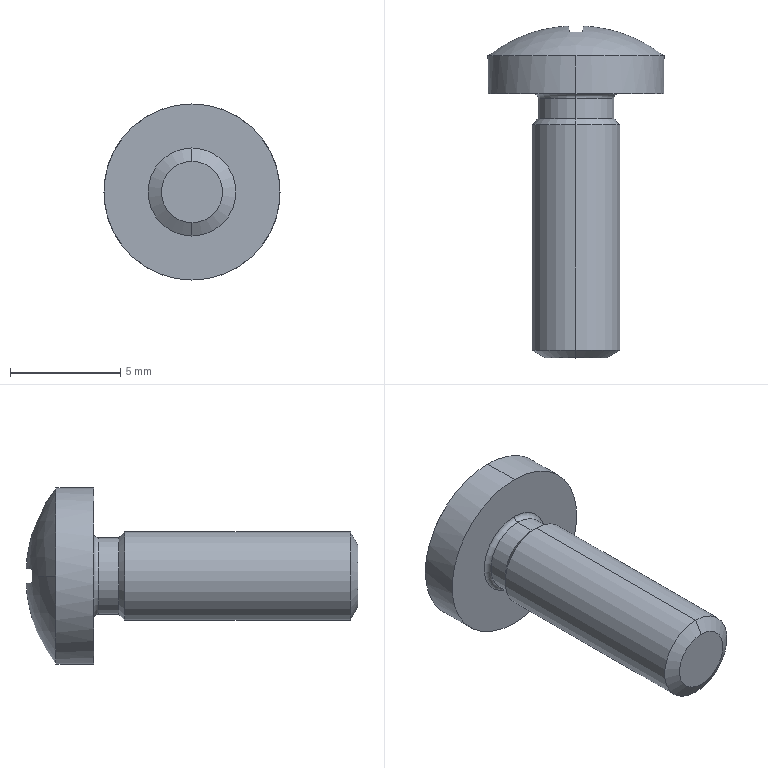Component | SolidWorks | GB_T818-2000PhillipsPanHeadScrewM4_12-1 | 1 solid | 28 faces | box 8 x 15.08 x 8 mm | volume 264 mm3 | plane 14 | cylinder 6 | cone 4 | torus 2 | sphere 2 | commonest cylinder face diameters 3.464 x2 8 x2 4 x2
build123d program:
from build123d import *


with BuildPart() as part:
    # Sketch2 → Base-Revolve (revolve)
    with BuildSketch(Plane.XY, mode=Mode.PRIVATE) as base_revolve_sk:
        with BuildLine():
            Line((0, 0), (15.1, 0))
            Line((15.1, 0), (15.1, 2))
            Line((15.1, 2), (4.5, 2))
            Line((4.5, 2), (4.232, 1.732))
            Line((4.232, 1.732), (3.318, 1.732))
            ThreePointArc((3.318, 1.732), (3.164, 1.796), (3.1, 1.95))
            Line((3.1, 1.95), (3.1, 4))
            Line((3.1, 4), (1.377, 4))
            ThreePointArc((1.377, 4), (0.3538, 2.115), (0, 0))
        make_face()
    revolve(base_revolve_sk.sketch.rotate(Axis((-1.332, 0, 0), (1, 0, 0)), 90), axis=Axis((-1.332, 0, 0), (1, 0, 0)))

    # Sketch3 → Cut-Revolve1 (revolve, cut)
    with BuildSketch(Plane.XY, mode=Mode.PRIVATE) as cut_revolve1_sk:
        Polygon((14.754, 2), (15.454, 2), (15.1, 1.394), align=None)
    revolve(cut_revolve1_sk.sketch.rotate(Axis((-0.2428, 0, 0), (1, 0, 0)), 90), axis=Axis((-0.2428, 0, 0), (1, 0, 0)), mode=Mode.SUBTRACT)

    # Sketch5 → Cut-Loft1 section 0
    with BuildSketch(Plane(origin=(0, 0, 0), x_dir=(0, 0, -1), z_dir=(1, 0, 0)), mode=Mode.PRIVATE) as cut_loft1_s0:
        with BuildLine():
            Line((0.35, 2.2), (-0.35, 2.2))
            Line((-0.35, 2.2), (-0.35, -2.2))
            Line((-0.35, -2.2), (0.35, -2.2))
            Line((0.35, -2.2), (0.35, 2.2))
        make_face()
    cut_loft1 = loft([Vertex(2.4, 0, 0), cut_loft1_s0.sketch], mode=Mode.SUBTRACT)

    # Mirror1: Cut-Loft1 across plane
    add(cut_loft1.mirror(Plane(origin=(0, 0, 0), x_dir=(0, 0.7071, 0.7071), z_dir=(0, -0.7071, 0.7071))), mode=Mode.SUBTRACT)


solid = part.part

# Placed as in the assembly
solid = solid.moved(Location((-112.444, 119.266, -150.597), (0, 0, -90)))
STEP:
#1=COLOUR_RGB('',0.7922,0.8196,0.9333);
#2=FILL_AREA_STYLE_COLOUR('',#1);
#3=FILL_AREA_STYLE('',(#2));
#4=SURFACE_STYLE_FILL_AREA(#3);
#5=SURFACE_SIDE_STYLE('',(#4));
#6=SURFACE_STYLE_USAGE(.BOTH.,#5);
#7=PRESENTATION_STYLE_ASSIGNMENT((#6));
#8=CARTESIAN_POINT('',(-4.427,4.101,-5.874));
#9=VERTEX_POINT('',#8);
#10=CARTESIAN_POINT('',(-4.427,4.101,-5.984));
#11=VERTEX_POINT('',#10);
#12=CARTESIAN_POINT('',(-4.427,4.101,-5.929));
#13=DIRECTION('',(0.,1.,0.));
#14=DIRECTION('',(0.,0.,1.));
#15=AXIS2_PLACEMENT_3D('',#12,#13,#14);
#16=CIRCLE('',#15,0.05487);
#17=EDGE_CURVE('',#9,#11,#16,.T.);
#18=ORIENTED_EDGE('',*,*,#17,.T.);
#19=CARTESIAN_POINT('',(-4.427,4.115,-6.008));
#20=VERTEX_POINT('',#19);
#21=CARTESIAN_POINT('',(-4.427,4.115,-6.008));
#22=DIRECTION('',(0.,0.4959,-0.8684));
#23=VECTOR('',#22,39.37);
#24=LINE('',#21,#23);
#25=EDGE_CURVE('',#11,#20,#24,.T.);
#26=ORIENTED_EDGE('',*,*,#25,.T.);
#27=CARTESIAN_POINT('',(-4.427,4.115,-5.85));
#28=VERTEX_POINT('',#27);
#29=CARTESIAN_POINT('',(-4.427,4.115,-5.929));
#30=DIRECTION('',(0.,1.,0.));
#31=DIRECTION('',(0.,0.,1.));
#32=AXIS2_PLACEMENT_3D('',#29,#30,#31);
#33=CIRCLE('',#32,0.07874);
#34=EDGE_CURVE('',#28,#20,#33,.T.);
#35=ORIENTED_EDGE('',*,*,#34,.F.);
#36=CARTESIAN_POINT('',(-4.427,4.115,-5.85));
#37=DIRECTION('',(0.,0.4959,0.8684));
#38=VECTOR('',#37,39.37);
#39=LINE('',#36,#38);
#40=EDGE_CURVE('',#9,#28,#39,.T.);
#41=ORIENTED_EDGE('',*,*,#40,.F.);
#42=EDGE_LOOP('',(#18,#26,#35,#41));
#43=FACE_OUTER_BOUND('',#42,.T.);
#44=CARTESIAN_POINT('',(-4.427,4.115,-5.929));
#45=DIRECTION('',(0.,1.,0.));
#46=DIRECTION('',(0.,0.,1.));
#47=AXIS2_PLACEMENT_3D('',#44,#45,#46);
#48=CONICAL_SURFACE('',#47,0.07874,1.052);
#49=ADVANCED_FACE('',(#43),#48,.T.);
#50=CARTESIAN_POINT('',(-4.427,4.529,-5.861));
#51=VERTEX_POINT('',#50);
#52=CARTESIAN_POINT('',(-4.427,4.529,-5.997));
#53=VERTEX_POINT('',#52);
#54=CARTESIAN_POINT('',(-4.427,4.529,-5.929));
#55=DIRECTION('',(0.,1.,0.));
#56=DIRECTION('',(0.,0.,1.));
#57=AXIS2_PLACEMENT_3D('',#54,#55,#56);
#58=CIRCLE('',#57,0.06819);
#59=EDGE_CURVE('',#51,#53,#58,.T.);
#60=ORIENTED_EDGE('',*,*,#59,.F.);
#61=CARTESIAN_POINT('',(-4.427,4.518,-5.85));
#62=VERTEX_POINT('',#61);
#63=CARTESIAN_POINT('',(-4.427,4.518,-5.85));
#64=DIRECTION('',(0.,-0.7071,0.7071));
#65=VECTOR('',#64,39.37);
#66=LINE('',#63,#65);
#67=EDGE_CURVE('',#51,#62,#66,.T.);
#68=ORIENTED_EDGE('',*,*,#67,.T.);
#69=CARTESIAN_POINT('',(-4.427,4.518,-6.008));
#70=VERTEX_POINT('',#69);
#71=CARTESIAN_POINT('',(-4.427,4.518,-5.929));
#72=DIRECTION('',(0.,1.,0.));
#73=DIRECTION('',(0.,0.,1.));
#74=AXIS2_PLACEMENT_3D('',#71,#72,#73);
#75=CIRCLE('',#74,0.07874);
#76=EDGE_CURVE('',#62,#70,#75,.T.);
#77=ORIENTED_EDGE('',*,*,#76,.T.);
#78=CARTESIAN_POINT('',(-4.427,4.518,-6.008));
#79=DIRECTION('',(0.,-0.7071,-0.7071));
#80=VECTOR('',#79,39.37);
#81=LINE('',#78,#80);
#82=EDGE_CURVE('',#53,#70,#81,.T.);
#83=ORIENTED_EDGE('',*,*,#82,.F.);
#84=EDGE_LOOP('',(#60,#68,#77,#83));
#85=FACE_OUTER_BOUND('',#84,.T.);
#86=CARTESIAN_POINT('',(-4.427,4.518,-5.929));
#87=DIRECTION('',(0.,-1.,0.));
#88=DIRECTION('',(0.,0.,-1.));
#89=AXIS2_PLACEMENT_3D('',#86,#87,#88);
#90=CONICAL_SURFACE('',#89,0.07874,0.7854);
#91=ADVANCED_FACE('',(#85),#90,.T.);
#92=ORIENTED_EDGE('',*,*,#59,.T.);
#93=CARTESIAN_POINT('',(-4.427,4.565,-5.997));
#94=VERTEX_POINT('',#93);
#95=CARTESIAN_POINT('',(-4.427,4.748,-5.997));
#96=DIRECTION('',(0.,1.,0.));
#97=VECTOR('',#96,39.37);
#98=LINE('',#95,#97);
#99=EDGE_CURVE('',#53,#94,#98,.T.);
#100=ORIENTED_EDGE('',*,*,#99,.T.);
#101=CARTESIAN_POINT('',(-4.427,4.565,-5.861));
#102=VERTEX_POINT('',#101);
#103=CARTESIAN_POINT('',(-4.427,4.565,-5.929));
#104=DIRECTION('',(0.,1.,0.));
#105=DIRECTION('',(0.,0.,1.));
#106=AXIS2_PLACEMENT_3D('',#103,#104,#105);
#107=CIRCLE('',#106,0.06819);
#108=EDGE_CURVE('',#102,#94,#107,.T.);
#109=ORIENTED_EDGE('',*,*,#108,.F.);
#110=CARTESIAN_POINT('',(-4.427,4.748,-5.861));
#111=DIRECTION('',(0.,1.,0.));
#112=VECTOR('',#111,39.37);
#113=LINE('',#110,#112);
#114=EDGE_CURVE('',#51,#102,#113,.T.);
#115=ORIENTED_EDGE('',*,*,#114,.F.);
#116=EDGE_LOOP('',(#92,#100,#109,#115));
#117=FACE_OUTER_BOUND('',#116,.T.);
#118=CARTESIAN_POINT('',(-4.427,4.748,-5.929));
#119=DIRECTION('',(0.,1.,0.));
#120=DIRECTION('',(0.,0.,1.));
#121=AXIS2_PLACEMENT_3D('',#118,#119,#120);
#122=CYLINDRICAL_SURFACE('',#121,0.06819);
#123=ADVANCED_FACE('',(#117),#122,.T.);
#124=CARTESIAN_POINT('',(-4.427,4.573,-6.006));
#125=VERTEX_POINT('',#124);
#126=CARTESIAN_POINT('',(-4.427,4.573,-5.852));
#127=VERTEX_POINT('',#126);
#128=CARTESIAN_POINT('',(-4.427,4.573,-5.929));
#129=DIRECTION('',(0.,1.,0.));
#130=DIRECTION('',(0.,0.,1.));
#131=AXIS2_PLACEMENT_3D('',#128,#129,#130);
#132=CIRCLE('',#131,0.07677);
#133=EDGE_CURVE('',#125,#127,#132,.T.);
#134=ORIENTED_EDGE('',*,*,#133,.F.);
#135=CARTESIAN_POINT('',(-4.427,4.565,-6.006));
#136=DIRECTION('',(1.,0.,0.));
#137=DIRECTION('',(0.,0.,-1.));
#138=AXIS2_PLACEMENT_3D('',#135,#136,#137);
#139=CIRCLE('',#138,0.008583);
#140=EDGE_CURVE('',#125,#94,#139,.T.);
#141=ORIENTED_EDGE('',*,*,#140,.T.);
#142=CARTESIAN_POINT('',(-4.427,4.565,-5.929));
#143=DIRECTION('',(0.,1.,0.));
#144=DIRECTION('',(0.,0.,1.));
#145=AXIS2_PLACEMENT_3D('',#142,#143,#144);
#146=CIRCLE('',#145,0.06819);
#147=EDGE_CURVE('',#94,#102,#146,.T.);
#148=ORIENTED_EDGE('',*,*,#147,.T.);
#149=CARTESIAN_POINT('',(-4.427,4.565,-5.852));
#150=DIRECTION('',(-1.,0.,0.));
#151=DIRECTION('',(0.,0.,1.));
#152=AXIS2_PLACEMENT_3D('',#149,#150,#151);
#153=CIRCLE('',#152,0.008583);
#154=EDGE_CURVE('',#127,#102,#153,.T.);
#155=ORIENTED_EDGE('',*,*,#154,.F.);
#156=EDGE_LOOP('',(#134,#141,#148,#155));
#157=FACE_OUTER_BOUND('',#156,.T.);
#158=CARTESIAN_POINT('',(-4.427,4.565,-5.929));
#159=DIRECTION('',(0.,1.,0.));
#160=DIRECTION('',(0.,0.,1.));
#161=AXIS2_PLACEMENT_3D('',#158,#159,#160);
#162=TOROIDAL_SURFACE('',#161,0.07677,0.008583);
#163=ADVANCED_FACE('',(#157),#162,.F.);
#164=CARTESIAN_POINT('',(-4.427,4.573,-5.772));
#165=VERTEX_POINT('',#164);
#166=CARTESIAN_POINT('',(-4.427,4.573,-6.087));
#167=VERTEX_POINT('',#166);
#168=CARTESIAN_POINT('',(-4.427,4.573,-5.929));
#169=DIRECTION('',(0.,1.,0.));
#170=DIRECTION('',(0.,0.,1.));
#171=AXIS2_PLACEMENT_3D('',#168,#169,#170);
#172=CIRCLE('',#171,0.1575);
#173=EDGE_CURVE('',#165,#167,#172,.T.);
#174=ORIENTED_EDGE('',*,*,#173,.T.);
#175=CARTESIAN_POINT('',(-4.427,4.641,-6.087));
#176=VERTEX_POINT('',#175);
#177=CARTESIAN_POINT('',(-4.427,4.748,-6.087));
#178=DIRECTION('',(0.,1.,0.));
#179=VECTOR('',#178,39.37);
#180=LINE('',#177,#179);
#181=EDGE_CURVE('',#167,#176,#180,.T.);
#182=ORIENTED_EDGE('',*,*,#181,.T.);
#183=CARTESIAN_POINT('',(-4.269,4.641,-5.929));
#184=VERTEX_POINT('',#183);
#185=CARTESIAN_POINT('',(-4.427,4.641,-5.929));
#186=DIRECTION('',(0.,1.,0.));
#187=DIRECTION('',(0.,0.,1.));
#188=AXIS2_PLACEMENT_3D('',#185,#186,#187);
#189=CIRCLE('',#188,0.1575);
#190=EDGE_CURVE('',#184,#176,#189,.T.);
#191=ORIENTED_EDGE('',*,*,#190,.F.);
#192=CARTESIAN_POINT('',(-4.427,4.641,-5.772));
#193=VERTEX_POINT('',#192);
#194=CARTESIAN_POINT('',(-4.427,4.641,-5.929));
#195=DIRECTION('',(0.,1.,0.));
#196=DIRECTION('',(0.,0.,1.));
#197=AXIS2_PLACEMENT_3D('',#194,#195,#196);
#198=CIRCLE('',#197,0.1575);
#199=EDGE_CURVE('',#193,#184,#198,.T.);
#200=ORIENTED_EDGE('',*,*,#199,.F.);
#201=CARTESIAN_POINT('',(-4.427,4.748,-5.772));
#202=DIRECTION('',(0.,1.,0.));
#203=VECTOR('',#202,39.37);
#204=LINE('',#201,#203);
#205=EDGE_CURVE('',#165,#193,#204,.T.);
#206=ORIENTED_EDGE('',*,*,#205,.F.);
#207=EDGE_LOOP('',(#174,#182,#191,#200,#206));
#208=FACE_OUTER_BOUND('',#207,.T.);
#209=CARTESIAN_POINT('',(-4.427,4.748,-5.929));
#210=DIRECTION('',(0.,1.,0.));
#211=DIRECTION('',(0.,0.,1.));
#212=AXIS2_PLACEMENT_3D('',#209,#210,#211);
#213=CYLINDRICAL_SURFACE('',#212,0.1575);
#214=ADVANCED_FACE('',(#208),#213,.T.);
#215=ORIENTED_EDGE('',*,*,#190,.T.);
#216=CARTESIAN_POINT('',(-4.584,4.641,-5.929));
#217=VERTEX_POINT('',#216);
#218=CARTESIAN_POINT('',(-4.427,4.641,-5.929));
#219=DIRECTION('',(0.,1.,0.));
#220=DIRECTION('',(0.,0.,1.));
#221=AXIS2_PLACEMENT_3D('',#218,#219,#220);
#222=CIRCLE('',#221,0.1575);
#223=EDGE_CURVE('',#176,#217,#222,.T.);
#224=ORIENTED_EDGE('',*,*,#223,.T.);
#225=CARTESIAN_POINT('',(-4.503,4.684,-5.929));
#226=VERTEX_POINT('',#225);
#227=CARTESIAN_POINT('',(-4.427,4.44,-5.929));
#228=DIRECTION('',(0.,0.,-1.));
#229=DIRECTION('',(-1.,0.,0.));
#230=AXIS2_PLACEMENT_3D('',#227,#228,#229);
#231=CIRCLE('',#230,0.2559);
#232=EDGE_CURVE('',#217,#226,#231,.T.);
#233=ORIENTED_EDGE('',*,*,#232,.T.);
#234=CARTESIAN_POINT('',(-4.503,4.684,-5.941));
#235=VERTEX_POINT('',#234);
#236=CARTESIAN_POINT('',(-4.347,4.513,-5.929));
#237=DIRECTION('',(-0.7372,-0.6757,0.));
#238=DIRECTION('',(0.6757,-0.7372,0.));
#239=AXIS2_PLACEMENT_3D('',#236,#237,#238);
#240=CIRCLE('',#239,0.2315);
#241=EDGE_CURVE('',#226,#235,#240,.T.);
#242=ORIENTED_EDGE('',*,*,#241,.T.);
#243=CARTESIAN_POINT('',(-4.441,4.695,-5.943));
#244=VERTEX_POINT('',#243);
#245=CARTESIAN_POINT('',(-4.427,4.443,-5.906));
#246=DIRECTION('',(0.,-0.1443,-0.9895));
#247=DIRECTION('',(0.,0.9895,-0.1443));
#248=AXIS2_PLACEMENT_3D('',#245,#246,#247);
#249=CIRCLE('',#248,0.2548);
#250=EDGE_CURVE('',#235,#244,#249,.T.);
#251=ORIENTED_EDGE('',*,*,#250,.T.);
#252=CARTESIAN_POINT('',(-4.439,4.684,-6.005));
#253=VERTEX_POINT('',#252);
#254=CARTESIAN_POINT('',(-4.404,4.443,-5.929));
#255=DIRECTION('',(-0.9895,-0.1443,-0.));
#256=DIRECTION('',(0.1443,-0.9895,0.));
#257=AXIS2_PLACEMENT_3D('',#254,#255,#256);
#258=CIRCLE('',#257,0.2548);
#259=EDGE_CURVE('',#244,#253,#258,.T.);
#260=ORIENTED_EDGE('',*,*,#259,.T.);
#261=CARTESIAN_POINT('',(-4.415,4.684,-6.005));
#262=VERTEX_POINT('',#261);
#263=CARTESIAN_POINT('',(-4.427,4.513,-5.849));
#264=DIRECTION('',(0.,-0.6757,-0.7372));
#265=DIRECTION('',(0.,0.7372,-0.6757));
#266=AXIS2_PLACEMENT_3D('',#263,#264,#265);
#267=CIRCLE('',#266,0.2315);
#268=EDGE_CURVE('',#253,#262,#267,.T.);
#269=ORIENTED_EDGE('',*,*,#268,.T.);
#270=CARTESIAN_POINT('',(-4.413,4.695,-5.943));
#271=VERTEX_POINT('',#270);
#272=CARTESIAN_POINT('',(-4.45,4.443,-5.929));
#273=DIRECTION('',(0.9895,-0.1443,0.));
#274=DIRECTION('',(0.1443,0.9895,0.));
#275=AXIS2_PLACEMENT_3D('',#272,#273,#274);
#276=CIRCLE('',#275,0.2548);
#277=EDGE_CURVE('',#262,#271,#276,.T.);
#278=ORIENTED_EDGE('',*,*,#277,.T.);
#279=CARTESIAN_POINT('',(-4.351,4.684,-5.941));
#280=VERTEX_POINT('',#279);
#281=CARTESIAN_POINT('',(-4.427,4.443,-5.906));
#282=DIRECTION('',(0.,-0.1443,-0.9895));
#283=DIRECTION('',(0.,0.9895,-0.1443));
#284=AXIS2_PLACEMENT_3D('',#281,#282,#283);
#285=CIRCLE('',#284,0.2548);
#286=EDGE_CURVE('',#271,#280,#285,.T.);
#287=ORIENTED_EDGE('',*,*,#286,.T.);
#288=CARTESIAN_POINT('',(-4.351,4.684,-5.929));
#289=VERTEX_POINT('',#288);
#290=CARTESIAN_POINT('',(-4.507,4.513,-5.929));
#291=DIRECTION('',(0.7372,-0.6757,0.));
#292=DIRECTION('',(0.6757,0.7372,0.));
#293=AXIS2_PLACEMENT_3D('',#290,#291,#292);
#294=CIRCLE('',#293,0.2315);
#295=EDGE_CURVE('',#280,#289,#294,.T.);
#296=ORIENTED_EDGE('',*,*,#295,.T.);
#297=CARTESIAN_POINT('',(-4.427,4.44,-5.929));
#298=DIRECTION('',(0.,0.,1.));
#299=DIRECTION('',(1.,0.,0.));
#300=AXIS2_PLACEMENT_3D('',#297,#298,#299);
#301=CIRCLE('',#300,0.2559);
#302=EDGE_CURVE('',#184,#289,#301,.T.);
#303=ORIENTED_EDGE('',*,*,#302,.F.);
#304=EDGE_LOOP('',(#215,#224,#233,#242,#251,#260,#269,#278,#287,#296,#303));
#305=FACE_OUTER_BOUND('',#304,.T.);
#306=CARTESIAN_POINT('',(-4.427,4.44,-5.929));
#307=DIRECTION('',(0.,0.,-1.));
#308=DIRECTION('',(1.,0.,0.));
#309=AXIS2_PLACEMENT_3D('',#306,#307,#308);
#310=SPHERICAL_SURFACE('',#309,0.2559);
#311=ADVANCED_FACE('',(#305),#310,.T.);
#312=ORIENTED_EDGE('',*,*,#34,.T.);
#313=CARTESIAN_POINT('',(-4.427,4.748,-6.008));
#314=DIRECTION('',(0.,1.,0.));
#315=VECTOR('',#314,39.37);
#316=LINE('',#313,#315);
#317=EDGE_CURVE('',#20,#70,#316,.T.);
#318=ORIENTED_EDGE('',*,*,#317,.T.);
#319=ORIENTED_EDGE('',*,*,#76,.F.);
#320=CARTESIAN_POINT('',(-4.427,4.748,-5.85));
#321=DIRECTION('',(0.,1.,0.));
#322=VECTOR('',#321,39.37);
#323=LINE('',#320,#322);
#324=EDGE_CURVE('',#28,#62,#323,.T.);
#325=ORIENTED_EDGE('',*,*,#324,.F.);
#326=EDGE_LOOP('',(#312,#318,#319,#325));
#327=FACE_OUTER_BOUND('',#326,.T.);
#328=CARTESIAN_POINT('',(-4.427,4.748,-5.929));
#329=DIRECTION('',(0.,1.,0.));
#330=DIRECTION('',(0.,0.,1.));
#331=AXIS2_PLACEMENT_3D('',#328,#329,#330);
#332=CYLINDRICAL_SURFACE('',#331,0.07874);
#333=ADVANCED_FACE('',(#327),#332,.T.);
#334=CARTESIAN_POINT('',(-4.427,4.601,-5.929));
#335=VERTEX_POINT('',#334);
#336=CARTESIAN_POINT('',(-4.427,4.601,-5.929));
#337=DIRECTION('',(-0.6719,0.7329,-0.1069));
#338=VECTOR('',#337,39.37);
#339=LINE('',#336,#338);
#340=EDGE_CURVE('',#335,#235,#339,.T.);
#341=ORIENTED_EDGE('',*,*,#340,.F.);
#342=CARTESIAN_POINT('',(-4.427,4.601,-5.929));
#343=DIRECTION('',(-0.1428,0.9794,-0.1428));
#344=VECTOR('',#343,39.37);
#345=LINE('',#342,#344);
#346=EDGE_CURVE('',#335,#244,#345,.T.);
#347=ORIENTED_EDGE('',*,*,#346,.T.);
#348=ORIENTED_EDGE('',*,*,#250,.F.);
#349=EDGE_LOOP('',(#341,#347,#348));
#350=FACE_OUTER_BOUND('',#349,.T.);
#351=CARTESIAN_POINT('',(-4.427,4.601,-5.929));
#352=DIRECTION('',(0.,-0.1443,-0.9895));
#353=DIRECTION('',(0.,0.9895,-0.1443));
#354=AXIS2_PLACEMENT_3D('',#351,#352,#353);
#355=PLANE('',#354);
#356=ADVANCED_FACE('',(#350),#355,.F.);
#357=CARTESIAN_POINT('',(-4.441,4.695,-5.915));
#358=VERTEX_POINT('',#357);
#359=CARTESIAN_POINT('',(-4.503,4.684,-5.917));
#360=VERTEX_POINT('',#359);
#361=CARTESIAN_POINT('',(-4.427,4.443,-5.952));
#362=DIRECTION('',(0.,-0.1443,0.9895));
#363=DIRECTION('',(0.,-0.9895,-0.1443));
#364=AXIS2_PLACEMENT_3D('',#361,#362,#363);
#365=CIRCLE('',#364,0.2548);
#366=EDGE_CURVE('',#358,#360,#365,.T.);
#367=ORIENTED_EDGE('',*,*,#366,.F.);
#368=CARTESIAN_POINT('',(-4.427,4.601,-5.929));
#369=DIRECTION('',(0.1428,-0.9794,-0.1428));
#370=VECTOR('',#369,39.37);
#371=LINE('',#368,#370);
#372=EDGE_CURVE('',#358,#335,#371,.T.);
#373=ORIENTED_EDGE('',*,*,#372,.T.);
#374=CARTESIAN_POINT('',(-4.427,4.601,-5.929));
#375=DIRECTION('',(-0.6719,0.7329,0.1069));
#376=VECTOR('',#375,39.37);
#377=LINE('',#374,#376);
#378=EDGE_CURVE('',#335,#360,#377,.T.);
#379=ORIENTED_EDGE('',*,*,#378,.T.);
#380=EDGE_LOOP('',(#367,#373,#379));
#381=FACE_OUTER_BOUND('',#380,.T.);
#382=CARTESIAN_POINT('',(-4.427,4.601,-5.929));
#383=DIRECTION('',(0.,-0.1443,0.9895));
#384=DIRECTION('',(0.,-0.9895,-0.1443));
#385=AXIS2_PLACEMENT_3D('',#382,#383,#384);
#386=PLANE('',#385);
#387=ADVANCED_FACE('',(#381),#386,.F.);
#388=ORIENTED_EDGE('',*,*,#317,.F.);
#389=CARTESIAN_POINT('',(-4.427,4.115,-5.929));
#390=DIRECTION('',(0.,1.,0.));
#391=DIRECTION('',(0.,0.,1.));
#392=AXIS2_PLACEMENT_3D('',#389,#390,#391);
#393=CIRCLE('',#392,0.07874);
#394=EDGE_CURVE('',#20,#28,#393,.T.);
#395=ORIENTED_EDGE('',*,*,#394,.T.);
#396=ORIENTED_EDGE('',*,*,#324,.T.);
#397=CARTESIAN_POINT('',(-4.427,4.518,-5.929));
#398=DIRECTION('',(0.,1.,0.));
#399=DIRECTION('',(0.,0.,1.));
#400=AXIS2_PLACEMENT_3D('',#397,#398,#399);
#401=CIRCLE('',#400,0.07874);
#402=EDGE_CURVE('',#70,#62,#401,.T.);
#403=ORIENTED_EDGE('',*,*,#402,.F.);
#404=EDGE_LOOP('',(#388,#395,#396,#403));
#405=FACE_OUTER_BOUND('',#404,.T.);
#406=CARTESIAN_POINT('',(-4.427,4.748,-5.929));
#407=DIRECTION('',(0.,1.,0.));
#408=DIRECTION('',(0.,0.,1.));
#409=AXIS2_PLACEMENT_3D('',#406,#407,#408);
#410=CYLINDRICAL_SURFACE('',#409,0.07874);
#411=ADVANCED_FACE('',(#405),#410,.T.);
#412=ORIENTED_EDGE('',*,*,#232,.F.);
#413=CARTESIAN_POINT('',(-4.427,4.641,-5.929));
#414=DIRECTION('',(0.,1.,0.));
#415=DIRECTION('',(0.,0.,1.));
#416=AXIS2_PLACEMENT_3D('',#413,#414,#415);
#417=CIRCLE('',#416,0.1575);
#418=EDGE_CURVE('',#217,#193,#417,.T.);
#419=ORIENTED_EDGE('',*,*,#418,.T.);
#420=ORIENTED_EDGE('',*,*,#199,.T.);
#421=ORIENTED_EDGE('',*,*,#302,.T.);
#422=CARTESIAN_POINT('',(-4.351,4.684,-5.917));
#423=VERTEX_POINT('',#422);
#424=CARTESIAN_POINT('',(-4.507,4.513,-5.929));
#425=DIRECTION('',(0.7372,-0.6757,0.));
#426=DIRECTION('',(0.6757,0.7372,0.));
#427=AXIS2_PLACEMENT_3D('',#424,#425,#426);
#428=CIRCLE('',#427,0.2315);
#429=EDGE_CURVE('',#289,#423,#428,.T.);
#430=ORIENTED_EDGE('',*,*,#429,.T.);
#431=CARTESIAN_POINT('',(-4.413,4.695,-5.915));
#432=VERTEX_POINT('',#431);
#433=CARTESIAN_POINT('',(-4.427,4.443,-5.952));
#434=DIRECTION('',(0.,-0.1443,0.9895));
#435=DIRECTION('',(0.,-0.9895,-0.1443));
#436=AXIS2_PLACEMENT_3D('',#433,#434,#435);
#437=CIRCLE('',#436,0.2548);
#438=EDGE_CURVE('',#423,#432,#437,.T.);
#439=ORIENTED_EDGE('',*,*,#438,.T.);
#440=CARTESIAN_POINT('',(-4.415,4.684,-5.853));
#441=VERTEX_POINT('',#440);
#442=CARTESIAN_POINT('',(-4.45,4.443,-5.929));
#443=DIRECTION('',(0.9895,-0.1443,0.));
#444=DIRECTION('',(0.1443,0.9895,0.));
#445=AXIS2_PLACEMENT_3D('',#442,#443,#444);
#446=CIRCLE('',#445,0.2548);
#447=EDGE_CURVE('',#432,#441,#446,.T.);
#448=ORIENTED_EDGE('',*,*,#447,.T.);
#449=CARTESIAN_POINT('',(-4.439,4.684,-5.853));
#450=VERTEX_POINT('',#449);
#451=CARTESIAN_POINT('',(-4.427,4.513,-6.009));
#452=DIRECTION('',(-0.,-0.6757,0.7372));
#453=DIRECTION('',(0.,-0.7372,-0.6757));
#454=AXIS2_PLACEMENT_3D('',#451,#452,#453);
#455=CIRCLE('',#454,0.2315);
#456=EDGE_CURVE('',#441,#450,#455,.T.);
#457=ORIENTED_EDGE('',*,*,#456,.T.);
#458=CARTESIAN_POINT('',(-4.404,4.443,-5.929));
#459=DIRECTION('',(-0.9895,-0.1443,-0.));
#460=DIRECTION('',(0.1443,-0.9895,0.));
#461=AXIS2_PLACEMENT_3D('',#458,#459,#460);
#462=CIRCLE('',#461,0.2548);
#463=EDGE_CURVE('',#450,#358,#462,.T.);
#464=ORIENTED_EDGE('',*,*,#463,.T.);
#465=ORIENTED_EDGE('',*,*,#366,.T.);
#466=CARTESIAN_POINT('',(-4.347,4.513,-5.929));
#467=DIRECTION('',(-0.7372,-0.6757,0.));
#468=DIRECTION('',(0.6757,-0.7372,0.));
#469=AXIS2_PLACEMENT_3D('',#466,#467,#468);
#470=CIRCLE('',#469,0.2315);
#471=EDGE_CURVE('',#360,#226,#470,.T.);
#472=ORIENTED_EDGE('',*,*,#471,.T.);
#473=EDGE_LOOP('',(#412,#419,#420,#421,#430,#439,#448,#457,#464,#465,#472));
#474=FACE_OUTER_BOUND('',#473,.T.);
#475=CARTESIAN_POINT('',(-4.427,4.44,-5.929));
#476=DIRECTION('',(0.,0.,-1.));
#477=DIRECTION('',(1.,0.,0.));
#478=AXIS2_PLACEMENT_3D('',#475,#476,#477);
#479=SPHERICAL_SURFACE('',#478,0.2559);
#480=ADVANCED_FACE('',(#474),#479,.T.);
#481=ORIENTED_EDGE('',*,*,#181,.F.);
#482=CARTESIAN_POINT('',(-4.427,4.573,-5.929));
#483=DIRECTION('',(0.,1.,0.));
#484=DIRECTION('',(0.,0.,1.));
#485=AXIS2_PLACEMENT_3D('',#482,#483,#484);
#486=CIRCLE('',#485,0.1575);
#487=EDGE_CURVE('',#167,#165,#486,.T.);
#488=ORIENTED_EDGE('',*,*,#487,.T.);
#489=ORIENTED_EDGE('',*,*,#205,.T.);
#490=ORIENTED_EDGE('',*,*,#418,.F.);
#491=ORIENTED_EDGE('',*,*,#223,.F.);
#492=EDGE_LOOP('',(#481,#488,#489,#490,#491));
#493=FACE_OUTER_BOUND('',#492,.T.);
#494=CARTESIAN_POINT('',(-4.427,4.748,-5.929));
#495=DIRECTION('',(0.,1.,0.));
#496=DIRECTION('',(0.,0.,1.));
#497=AXIS2_PLACEMENT_3D('',#494,#495,#496);
#498=CYLINDRICAL_SURFACE('',#497,0.1575);
#499=ADVANCED_FACE('',(#493),#498,.T.);
#500=ORIENTED_EDGE('',*,*,#173,.F.);
#501=ORIENTED_EDGE('',*,*,#487,.F.);
#502=EDGE_LOOP('',(#500,#501));
#503=FACE_OUTER_BOUND('',#502,.T.);
#504=CARTESIAN_POINT('',(-4.427,4.573,-5.929));
#505=DIRECTION('',(0.,1.,0.));
#506=DIRECTION('',(0.,0.,1.));
#507=AXIS2_PLACEMENT_3D('',#504,#505,#506);
#508=CIRCLE('',#507,0.07677);
#509=EDGE_CURVE('',#127,#125,#508,.T.);
#510=ORIENTED_EDGE('',*,*,#509,.T.);
#511=ORIENTED_EDGE('',*,*,#133,.T.);
#512=EDGE_LOOP('',(#510,#511));
#513=FACE_BOUND('',#512,.T.);
#514=CARTESIAN_POINT('',(-4.35,4.573,-5.929));
#515=DIRECTION('',(0.,1.,0.));
#516=DIRECTION('',(0.,0.,1.));
#517=AXIS2_PLACEMENT_3D('',#514,#515,#516);
#518=PLANE('',#517);
#519=ADVANCED_FACE('',(#503,#513),#518,.F.);
#520=ORIENTED_EDGE('',*,*,#140,.F.);
#521=ORIENTED_EDGE('',*,*,#509,.F.);
#522=ORIENTED_EDGE('',*,*,#154,.T.);
#523=ORIENTED_EDGE('',*,*,#108,.T.);
#524=EDGE_LOOP('',(#520,#521,#522,#523));
#525=FACE_OUTER_BOUND('',#524,.T.);
#526=CARTESIAN_POINT('',(-4.427,4.565,-5.929));
#527=DIRECTION('',(0.,1.,0.));
#528=DIRECTION('',(0.,0.,1.));
#529=AXIS2_PLACEMENT_3D('',#526,#527,#528);
#530=TOROIDAL_SURFACE('',#529,0.07677,0.008583);
#531=ADVANCED_FACE('',(#525),#530,.F.);
#532=ORIENTED_EDGE('',*,*,#99,.F.);
#533=CARTESIAN_POINT('',(-4.427,4.529,-5.929));
#534=DIRECTION('',(0.,1.,0.));
#535=DIRECTION('',(0.,0.,1.));
#536=AXIS2_PLACEMENT_3D('',#533,#534,#535);
#537=CIRCLE('',#536,0.06819);
#538=EDGE_CURVE('',#53,#51,#537,.T.);
#539=ORIENTED_EDGE('',*,*,#538,.T.);
#540=ORIENTED_EDGE('',*,*,#114,.T.);
#541=ORIENTED_EDGE('',*,*,#147,.F.);
#542=EDGE_LOOP('',(#532,#539,#540,#541));
#543=FACE_OUTER_BOUND('',#542,.T.);
#544=CARTESIAN_POINT('',(-4.427,4.748,-5.929));
#545=DIRECTION('',(0.,1.,0.));
#546=DIRECTION('',(0.,0.,1.));
#547=AXIS2_PLACEMENT_3D('',#544,#545,#546);
#548=CYLINDRICAL_SURFACE('',#547,0.06819);
#549=ADVANCED_FACE('',(#543),#548,.T.);
#550=ORIENTED_EDGE('',*,*,#67,.F.);
#551=ORIENTED_EDGE('',*,*,#538,.F.);
#552=ORIENTED_EDGE('',*,*,#82,.T.);
#553=ORIENTED_EDGE('',*,*,#402,.T.);
#554=EDGE_LOOP('',(#550,#551,#552,#553));
#555=FACE_OUTER_BOUND('',#554,.T.);
#556=CARTESIAN_POINT('',(-4.427,4.518,-5.929));
#557=DIRECTION('',(0.,-1.,0.));
#558=DIRECTION('',(0.,0.,-1.));
#559=AXIS2_PLACEMENT_3D('',#556,#557,#558);
#560=CONICAL_SURFACE('',#559,0.07874,0.7854);
#561=ADVANCED_FACE('',(#555),#560,.T.);
#562=ORIENTED_EDGE('',*,*,#25,.F.);
#563=CARTESIAN_POINT('',(-4.427,4.101,-5.929));
#564=DIRECTION('',(0.,1.,0.));
#565=DIRECTION('',(0.,0.,1.));
#566=AXIS2_PLACEMENT_3D('',#563,#564,#565);
#567=CIRCLE('',#566,0.05487);
#568=EDGE_CURVE('',#11,#9,#567,.T.);
#569=ORIENTED_EDGE('',*,*,#568,.T.);
#570=ORIENTED_EDGE('',*,*,#40,.T.);
#571=ORIENTED_EDGE('',*,*,#394,.F.);
#572=EDGE_LOOP('',(#562,#569,#570,#571));
#573=FACE_OUTER_BOUND('',#572,.T.);
#574=CARTESIAN_POINT('',(-4.427,4.115,-5.929));
#575=DIRECTION('',(0.,1.,0.));
#576=DIRECTION('',(0.,0.,1.));
#577=AXIS2_PLACEMENT_3D('',#574,#575,#576);
#578=CONICAL_SURFACE('',#577,0.07874,1.052);
#579=ADVANCED_FACE('',(#573),#578,.T.);
#580=ORIENTED_EDGE('',*,*,#17,.F.);
#581=ORIENTED_EDGE('',*,*,#568,.F.);
#582=EDGE_LOOP('',(#580,#581));
#583=FACE_OUTER_BOUND('',#582,.T.);
#584=CARTESIAN_POINT('',(-4.427,4.101,-5.929));
#585=DIRECTION('',(0.,1.,0.));
#586=DIRECTION('',(0.,0.,1.));
#587=AXIS2_PLACEMENT_3D('',#584,#585,#586);
#588=PLANE('',#587);
#589=ADVANCED_FACE('',(#583),#588,.F.);
#590=ORIENTED_EDGE('',*,*,#286,.F.);
#591=CARTESIAN_POINT('',(-4.427,4.601,-5.929));
#592=DIRECTION('',(-0.1428,-0.9794,0.1428));
#593=VECTOR('',#592,39.37);
#594=LINE('',#591,#593);
#595=EDGE_CURVE('',#271,#335,#594,.T.);
#596=ORIENTED_EDGE('',*,*,#595,.T.);
#597=CARTESIAN_POINT('',(-4.427,4.601,-5.929));
#598=DIRECTION('',(0.6719,0.7329,-0.1069));
#599=VECTOR('',#598,39.37);
#600=LINE('',#597,#599);
#601=EDGE_CURVE('',#335,#280,#600,.T.);
#602=ORIENTED_EDGE('',*,*,#601,.T.);
#603=EDGE_LOOP('',(#590,#596,#602));
#604=FACE_OUTER_BOUND('',#603,.T.);
#605=CARTESIAN_POINT('',(-4.427,4.601,-5.929));
#606=DIRECTION('',(0.,-0.1443,-0.9895));
#607=DIRECTION('',(0.,0.9895,-0.1443));
#608=AXIS2_PLACEMENT_3D('',#605,#606,#607);
#609=PLANE('',#608);
#610=ADVANCED_FACE('',(#604),#609,.F.);
#611=ORIENTED_EDGE('',*,*,#601,.F.);
#612=CARTESIAN_POINT('',(-4.427,4.601,-5.929));
#613=DIRECTION('',(0.6719,0.7329,0.1069));
#614=VECTOR('',#613,39.37);
#615=LINE('',#612,#614);
#616=EDGE_CURVE('',#335,#423,#615,.T.);
#617=ORIENTED_EDGE('',*,*,#616,.T.);
#618=ORIENTED_EDGE('',*,*,#429,.F.);
#619=ORIENTED_EDGE('',*,*,#295,.F.);
#620=EDGE_LOOP('',(#611,#617,#618,#619));
#621=FACE_OUTER_BOUND('',#620,.T.);
#622=CARTESIAN_POINT('',(-4.34,4.696,-5.943));
#623=DIRECTION('',(0.7372,-0.6757,0.));
#624=DIRECTION('',(0.6757,0.7372,0.));
#625=AXIS2_PLACEMENT_3D('',#622,#623,#624);
#626=PLANE('',#625);
#627=ADVANCED_FACE('',(#621),#626,.F.);
#628=ORIENTED_EDGE('',*,*,#378,.F.);
#629=ORIENTED_EDGE('',*,*,#340,.T.);
#630=ORIENTED_EDGE('',*,*,#241,.F.);
#631=ORIENTED_EDGE('',*,*,#471,.F.);
#632=EDGE_LOOP('',(#628,#629,#630,#631));
#633=FACE_OUTER_BOUND('',#632,.T.);
#634=CARTESIAN_POINT('',(-4.514,4.696,-5.915));
#635=DIRECTION('',(-0.7372,-0.6757,0.));
#636=DIRECTION('',(0.6757,-0.7372,0.));
#637=AXIS2_PLACEMENT_3D('',#634,#635,#636);
#638=PLANE('',#637);
#639=ADVANCED_FACE('',(#633),#638,.F.);
#640=ORIENTED_EDGE('',*,*,#616,.F.);
#641=CARTESIAN_POINT('',(-4.427,4.601,-5.929));
#642=DIRECTION('',(0.1428,0.9794,0.1428));
#643=VECTOR('',#642,39.37);
#644=LINE('',#641,#643);
#645=EDGE_CURVE('',#335,#432,#644,.T.);
#646=ORIENTED_EDGE('',*,*,#645,.T.);
#647=ORIENTED_EDGE('',*,*,#438,.F.);
#648=EDGE_LOOP('',(#640,#646,#647));
#649=FACE_OUTER_BOUND('',#648,.T.);
#650=CARTESIAN_POINT('',(-4.427,4.601,-5.929));
#651=DIRECTION('',(0.,-0.1443,0.9895));
#652=DIRECTION('',(0.,-0.9895,-0.1443));
#653=AXIS2_PLACEMENT_3D('',#650,#651,#652);
#654=PLANE('',#653);
#655=ADVANCED_FACE('',(#649),#654,.F.);
#656=CARTESIAN_POINT('',(-4.427,4.601,-5.929));
#657=DIRECTION('',(-0.1069,0.7329,0.6719));
#658=VECTOR('',#657,39.37);
#659=LINE('',#656,#658);
#660=EDGE_CURVE('',#335,#450,#659,.T.);
#661=ORIENTED_EDGE('',*,*,#660,.F.);
#662=ORIENTED_EDGE('',*,*,#372,.F.);
#663=ORIENTED_EDGE('',*,*,#463,.F.);
#664=EDGE_LOOP('',(#661,#662,#663));
#665=FACE_OUTER_BOUND('',#664,.T.);
#666=CARTESIAN_POINT('',(-4.427,4.601,-5.929));
#667=DIRECTION('',(-0.9895,-0.1443,-0.));
#668=DIRECTION('',(-0.1443,0.9895,-0.));
#669=AXIS2_PLACEMENT_3D('',#666,#667,#668);
#670=PLANE('',#669);
#671=ADVANCED_FACE('',(#665),#670,.F.);
#672=ORIENTED_EDGE('',*,*,#645,.F.);
#673=CARTESIAN_POINT('',(-4.427,4.601,-5.929));
#674=DIRECTION('',(0.1069,0.7329,0.6719));
#675=VECTOR('',#674,39.37);
#676=LINE('',#673,#675);
#677=EDGE_CURVE('',#335,#441,#676,.T.);
#678=ORIENTED_EDGE('',*,*,#677,.T.);
#679=ORIENTED_EDGE('',*,*,#447,.F.);
#680=EDGE_LOOP('',(#672,#678,#679));
#681=FACE_OUTER_BOUND('',#680,.T.);
#682=CARTESIAN_POINT('',(-4.427,4.601,-5.929));
#683=DIRECTION('',(0.9895,-0.1443,0.));
#684=DIRECTION('',(-0.1443,-0.9895,-0.));
#685=AXIS2_PLACEMENT_3D('',#682,#683,#684);
#686=PLANE('',#685);
#687=ADVANCED_FACE('',(#681),#686,.F.);
#688=ORIENTED_EDGE('',*,*,#677,.F.);
#689=ORIENTED_EDGE('',*,*,#660,.T.);
#690=ORIENTED_EDGE('',*,*,#456,.F.);
#691=EDGE_LOOP('',(#688,#689,#690));
#692=FACE_OUTER_BOUND('',#691,.T.);
#693=CARTESIAN_POINT('',(-4.441,4.696,-5.842));
#694=DIRECTION('',(-0.,-0.6757,0.7372));
#695=DIRECTION('',(-0.,0.7372,0.6757));
#696=AXIS2_PLACEMENT_3D('',#693,#694,#695);
#697=PLANE('',#696);
#698=ADVANCED_FACE('',(#692),#697,.F.);
#699=ORIENTED_EDGE('',*,*,#346,.F.);
#700=CARTESIAN_POINT('',(-4.427,4.601,-5.929));
#701=DIRECTION('',(-0.1069,0.7329,-0.6719));
#702=VECTOR('',#701,39.37);
#703=LINE('',#700,#702);
#704=EDGE_CURVE('',#335,#253,#703,.T.);
#705=ORIENTED_EDGE('',*,*,#704,.T.);
#706=ORIENTED_EDGE('',*,*,#259,.F.);
#707=EDGE_LOOP('',(#699,#705,#706));
#708=FACE_OUTER_BOUND('',#707,.T.);
#709=CARTESIAN_POINT('',(-4.427,4.601,-5.929));
#710=DIRECTION('',(-0.9895,-0.1443,-0.));
#711=DIRECTION('',(-0.1443,0.9895,-0.));
#712=AXIS2_PLACEMENT_3D('',#709,#710,#711);
#713=PLANE('',#712);
#714=ADVANCED_FACE('',(#708),#713,.F.);
#715=ORIENTED_EDGE('',*,*,#704,.F.);
#716=CARTESIAN_POINT('',(-4.427,4.601,-5.929));
#717=DIRECTION('',(0.1069,0.7329,-0.6719));
#718=VECTOR('',#717,39.37);
#719=LINE('',#716,#718);
#720=EDGE_CURVE('',#335,#262,#719,.T.);
#721=ORIENTED_EDGE('',*,*,#720,.T.);
#722=ORIENTED_EDGE('',*,*,#268,.F.);
#723=EDGE_LOOP('',(#715,#721,#722));
#724=FACE_OUTER_BOUND('',#723,.T.);
#725=CARTESIAN_POINT('',(-4.413,4.696,-6.016));
#726=DIRECTION('',(0.,-0.6757,-0.7372));
#727=DIRECTION('',(-0.,-0.7372,0.6757));
#728=AXIS2_PLACEMENT_3D('',#725,#726,#727);
#729=PLANE('',#728);
#730=ADVANCED_FACE('',(#724),#729,.F.);
#731=ORIENTED_EDGE('',*,*,#720,.F.);
#732=ORIENTED_EDGE('',*,*,#595,.F.);
#733=ORIENTED_EDGE('',*,*,#277,.F.);
#734=EDGE_LOOP('',(#731,#732,#733));
#735=FACE_OUTER_BOUND('',#734,.T.);
#736=CARTESIAN_POINT('',(-4.427,4.601,-5.929));
#737=DIRECTION('',(0.9895,-0.1443,0.));
#738=DIRECTION('',(-0.1443,-0.9895,-0.));
#739=AXIS2_PLACEMENT_3D('',#736,#737,#738);
#740=PLANE('',#739);
#741=ADVANCED_FACE('',(#735),#740,.F.);
#742=CLOSED_SHELL('',(#49,#91,#123,#163,#214,#311,#333,#356,#387,#411,#480,#499,#519,#531,#549,#561,#579,#589,#610,#627,#639,#655,#671,#687,#698,#714,#730,#741));
#743=MANIFOLD_SOLID_BREP('',#742);
#744=STYLED_ITEM('',(#7),#743);
#745=PRESENTATION_LAYER_ASSIGNMENT('','',(#744));
#746=CARTESIAN_POINT('',(0.,0.,0.));
#747=DIRECTION('',(0.,0.,1.));
#748=DIRECTION('',(1.,0.,0.));
#749=AXIS2_PLACEMENT_3D('',#746,#747,#748);
#750=(LENGTH_UNIT()NAMED_UNIT(*)SI_UNIT($,.METRE.));
#751=LENGTH_MEASURE_WITH_UNIT(LENGTH_MEASURE(0.0254),#750);
#752=DIMENSIONAL_EXPONENTS(1.,0.,0.,0.,0.,0.,0.);
#753=(CONVERSION_BASED_UNIT('',#751)LENGTH_UNIT()NAMED_UNIT(#752));
#754=UNCERTAINTY_MEASURE_WITH_UNIT(LENGTH_MEASURE(0.00001),#753,'','');
#755=(NAMED_UNIT(*)PLANE_ANGLE_UNIT()SI_UNIT($,.RADIAN.));
#756=(NAMED_UNIT(*)SI_UNIT($,.STERADIAN.)SOLID_ANGLE_UNIT());
#757=(GEOMETRIC_REPRESENTATION_CONTEXT(3)GLOBAL_UNCERTAINTY_ASSIGNED_CONTEXT((#754))GLOBAL_UNIT_ASSIGNED_CONTEXT((#753,#755,#756))REPRESENTATION_CONTEXT('',''));
#758=ADVANCED_BREP_SHAPE_REPRESENTATION('',(#743,#749),#757);
#759=(LENGTH_UNIT()NAMED_UNIT(*)SI_UNIT($,.METRE.));
#760=LENGTH_MEASURE_WITH_UNIT(LENGTH_MEASURE(0.0254),#759);
#761=DIMENSIONAL_EXPONENTS(1.,0.,0.,0.,0.,0.,0.);
#762=(CONVERSION_BASED_UNIT('',#760)LENGTH_UNIT()NAMED_UNIT(#761));
#763=UNCERTAINTY_MEASURE_WITH_UNIT(LENGTH_MEASURE(0.00001),#762,'','');
#764=(NAMED_UNIT(*)PLANE_ANGLE_UNIT()SI_UNIT($,.RADIAN.));
#765=(NAMED_UNIT(*)SI_UNIT($,.STERADIAN.)SOLID_ANGLE_UNIT());
#766=(GEOMETRIC_REPRESENTATION_CONTEXT(3)GLOBAL_UNCERTAINTY_ASSIGNED_CONTEXT((#763))GLOBAL_UNIT_ASSIGNED_CONTEXT((#762,#764,#765))REPRESENTATION_CONTEXT('',''));
#767=MECHANICAL_DESIGN_GEOMETRIC_PRESENTATION_REPRESENTATION('',(#744),#766);